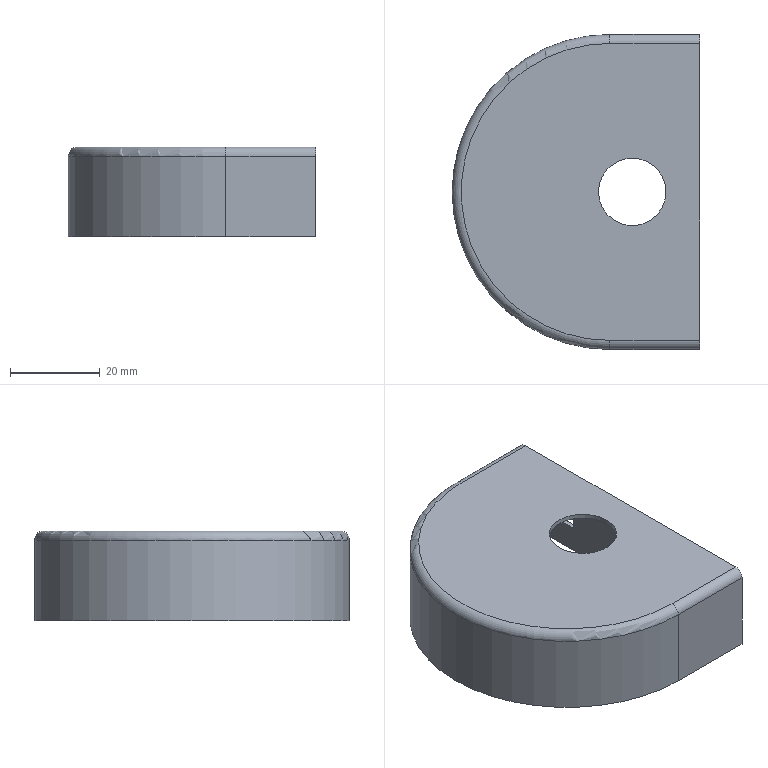Component | NX | LOCK_BODY_END_COVER | 1 solid | 31 faces | volume 11945 mm3 | plane 17 | cylinder 9 | cone 4 | torus 1 | commonest cylinder face diameters 3.5 x2 4 x2 70 x1 68 x1 15 x1 61.774 x1 44.045 x1